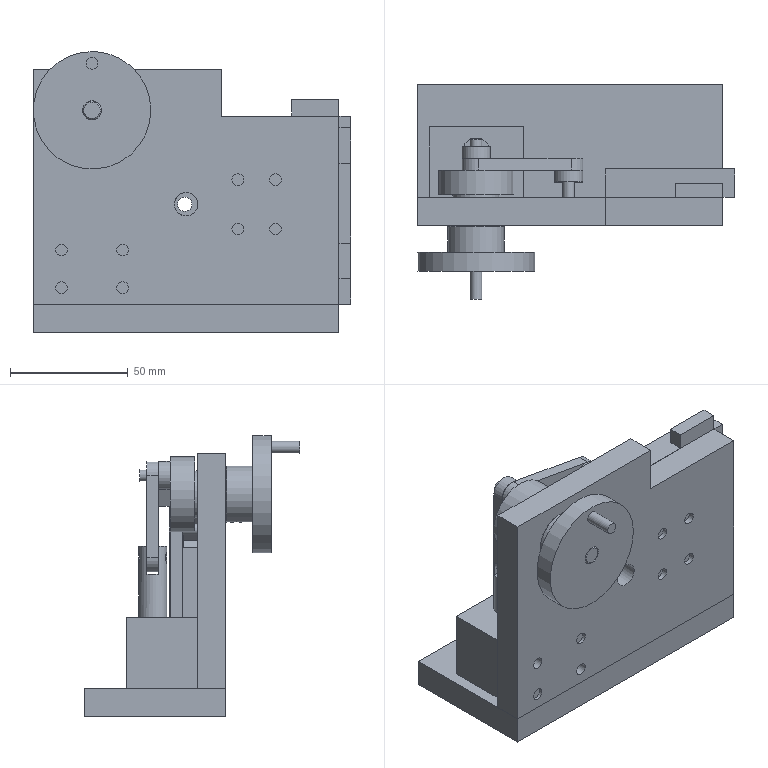Assembly | NX | mm | 25 component files | 25 solids | 246 faces | box 135 x 91.5 x 119.5 mm | volume 352094 mm3 | plane 162 | cylinder 78 | cone 6 | commonest cylinder face diameters 5 x34 12 x9 5.5 x8 10 x7 5.1 x6 8.28 x4 6.1 x2 8 x2
Bill of materials:
unnamed part 1 | 1 |  | Rectangular block-like plate with a stepped profile: a continuous back web carries three raised pads across one face (short top and bottom pads, a taller middle pad), with stepped notches on the opposite edge; four round holes in a 2x2 pattern pass through the middle pad region.
unnamed part 2 | 1 |  | Thin flat rectangular plate with two V-shaped (triangular) notches cut into one long edge; opposite edge straight.
unnamed part 3 | 6 |  | Plain solid circular cylinder (rod/pin blank) with flat ends.
unnamed part 4 | 2 |  | Stepped cylindrical pin: a longer smaller-diameter shank joined to a short larger-diameter head, with flat ends.
unnamed part 5 | 1 |  | Rectangular block with one larger round hole on the top face and four smaller round holes in a rectangular pattern on one side face.
unnamed part 6 | 1 |  | Circular flange disc with a smaller concentric cylindrical boss on one side; a central round through-hole and one smaller off-center hole near the rim.
unnamed part 7 | 3 |  | Solid circular cylinder (rod) with flat ends, relatively larger diameter-to-length ratio than a slender pin.
unnamed part 8 | 1 |  | Cylinder with a conical (pointed) top and a rectangular notch cut into the bottom edge of the cylindrical wall; the lower portion appears slightly reduced in diameter.
unnamed part 9 | 1 |  | Flat rectangular plate with a rectangular corner step cut out of one edge, two larger round holes and two groups of four smaller holes in square patterns.
unnamed part 10 | 1 |  | Cylindrical pin with a slot cut across one end forming two prongs, a cross hole passing through the prongs, and a slightly reduced diameter at the slotted end.
unnamed part 11 | 1 |  | Flat rectangular plate with one larger round hole near one end and two smaller round holes near one long edge.
unnamed part 12 | 1 |  | Thin elongated flat bar/link with one fully rounded end, a round hole near the rounded end, an elongated slot, a second round hole, and an open U-shaped slot at the opposite square end.
unnamed part 13 | 1 |  | Turned part shaped like a stepped shaft. A large, short cylindrical disc head is joined to a thin shoulder ring, then a medium-diameter shaft section, then a smaller-diameter end shaft with a chamfered tip. A small axial through-hole sits off-center in the disc.
unnamed part 14 | 1 |  | Flat, thin, elongated link/plate with fully rounded (obround) ends and one through-hole near each end. The hole at one end looks slightly larger than the hole at the other.
unnamed part 15 | 2 |  | Headed cylindrical pin: a long, plain, straight cylindrical shank with one short, larger-diameter cylindrical head. Both ends are flat.
unnamed part 16 | 1 |  | Flat elongated link/plate with fully rounded (obround) ends and two equal-size through-holes, one centered near each end. It is thicker relative to its width than unnamed part 14.
Mates:
1. touch align | groove_guide_block 1 face | vertical_plate 1 face
2. touch align | groove_guide_block 1 edge | vertical_plate 1 edge
3. concentric | groove_guide_block 1 edge | vertical_plate 1 edge
4. fix | vertical_plate 1 component
5. concentric | short_link 1 edge | slide_rod 1 edge
6. fix | round_guide_block 1 component
7. parallel | long_link 1 face | bi_link 1 face
8. concentric | long_link 1 edge | bi_link 1 edge
9. fix | eccentric_wheel 1 component
10. concentric | long_link 1 edge | eccentric_wheel 1 edge
11. touch align | handwheel 1 face | eccentric_wheel 1 face
12. concentric | eccentric_wheel 1 edge | handwheel 1 edge
13. touch align | M5x6 1 face | eccentric_wheel 1 face
14. distance | M5x6 1 face | eccentric_wheel 1 face
15. touch align | round_guide_block 1 face | hex_screw_M5_35 1 face
16. concentric | round_guide_block 1 edge | hex_screw_M5_35 1 edge
17. touch align | hex_screw_M5_35 2 face | round_guide_block 1 face
18. concentric | round_guide_block 1 edge | hex_screw_M5_35 2 edge
19. touch align | hex_screw_M5_16 2 face | groove_guide_block 1 face
20. touch align | hex_screw_M5_16 1 face | groove_guide_block 1 face
21. concentric | hex_screw_M5_16 2 edge | groove_guide_block 1 edge
22. concentric | hex_screw_M5_16 1 edge | groove_guide_block 1 edge
23. distance | vertical_plate 1 edge | dowel_pin_5_20 4 face
24. distance | dowel_pin_5_20 5 face | vertical_plate 1 face
25. touch align | vertical_plate 1 face | dowel_pin_5_20 3 face
26. touch align | vertical_plate 1 face | dowel_pin_5_20 2 face
27. concentric | dowel_pin_5_20 3 edge | round_guide_block 1 edge
28. concentric | dowel_pin_5_20 2 edge | round_guide_block 1 edge
29. touch align | dowel_pin_5_12 3 face | slide_rod 1 face
30. distance | short_link 1 face | dowel_pin_5_12 3 face
31. fix | bi_link 1 component
32. touch align | vertical_plate 1 face | V_slider 1 face
33. touch align | V_slider 1 face | groove_guide_block 1 face
34. distance | V_slider 1 face | groove_guide_block 1 face
35. concentric | dowel_pin_5_20 1 edge | handwheel 1 edge